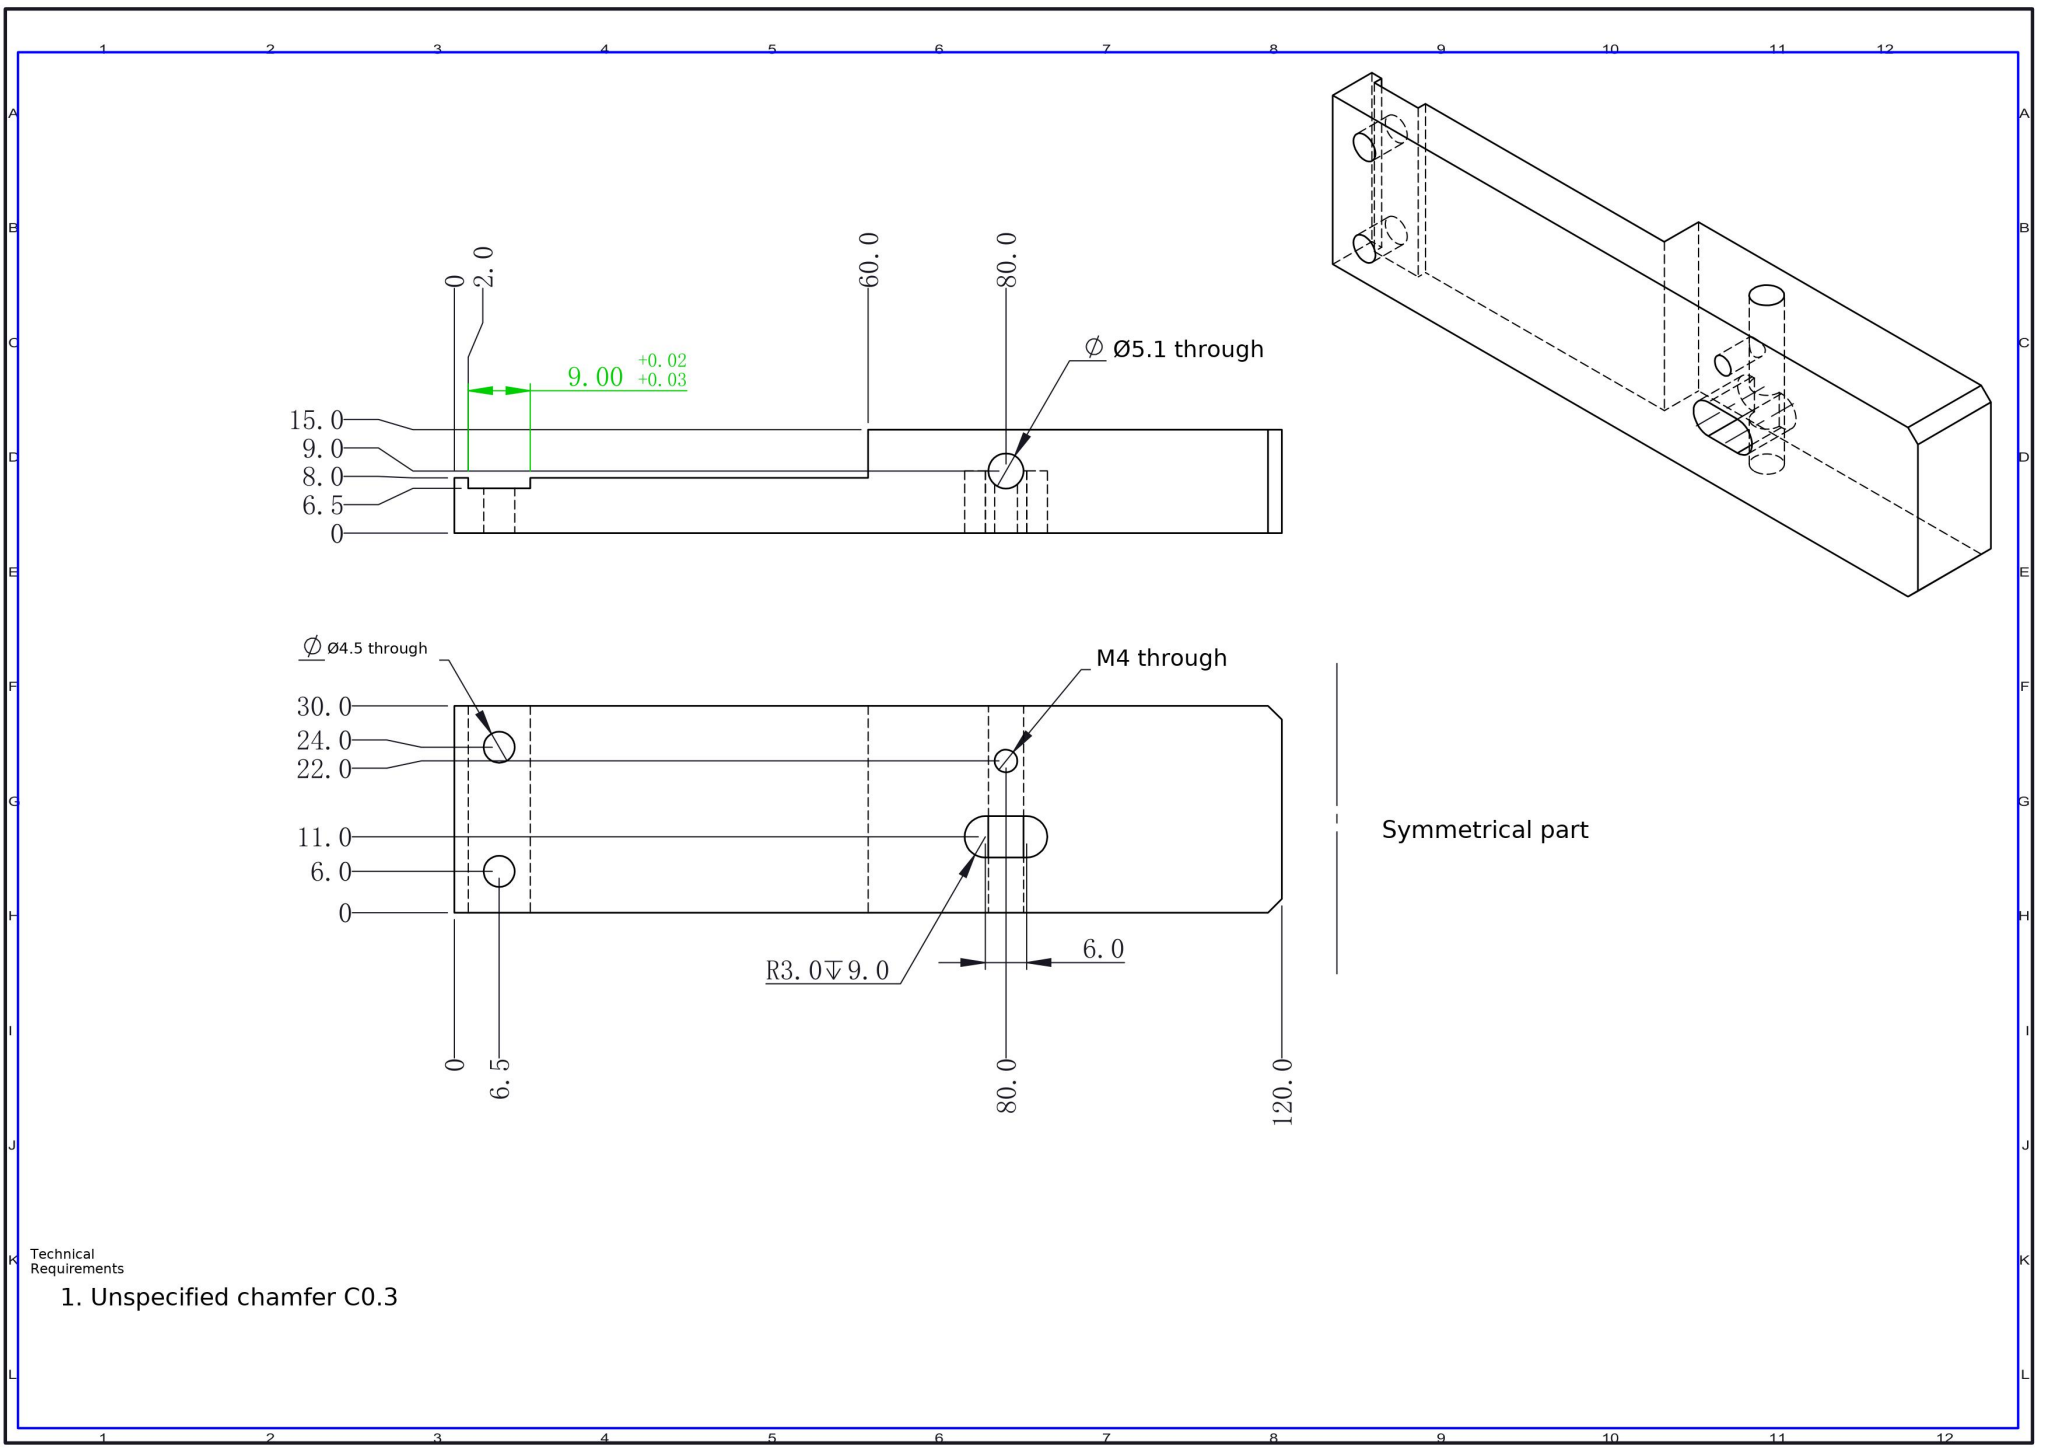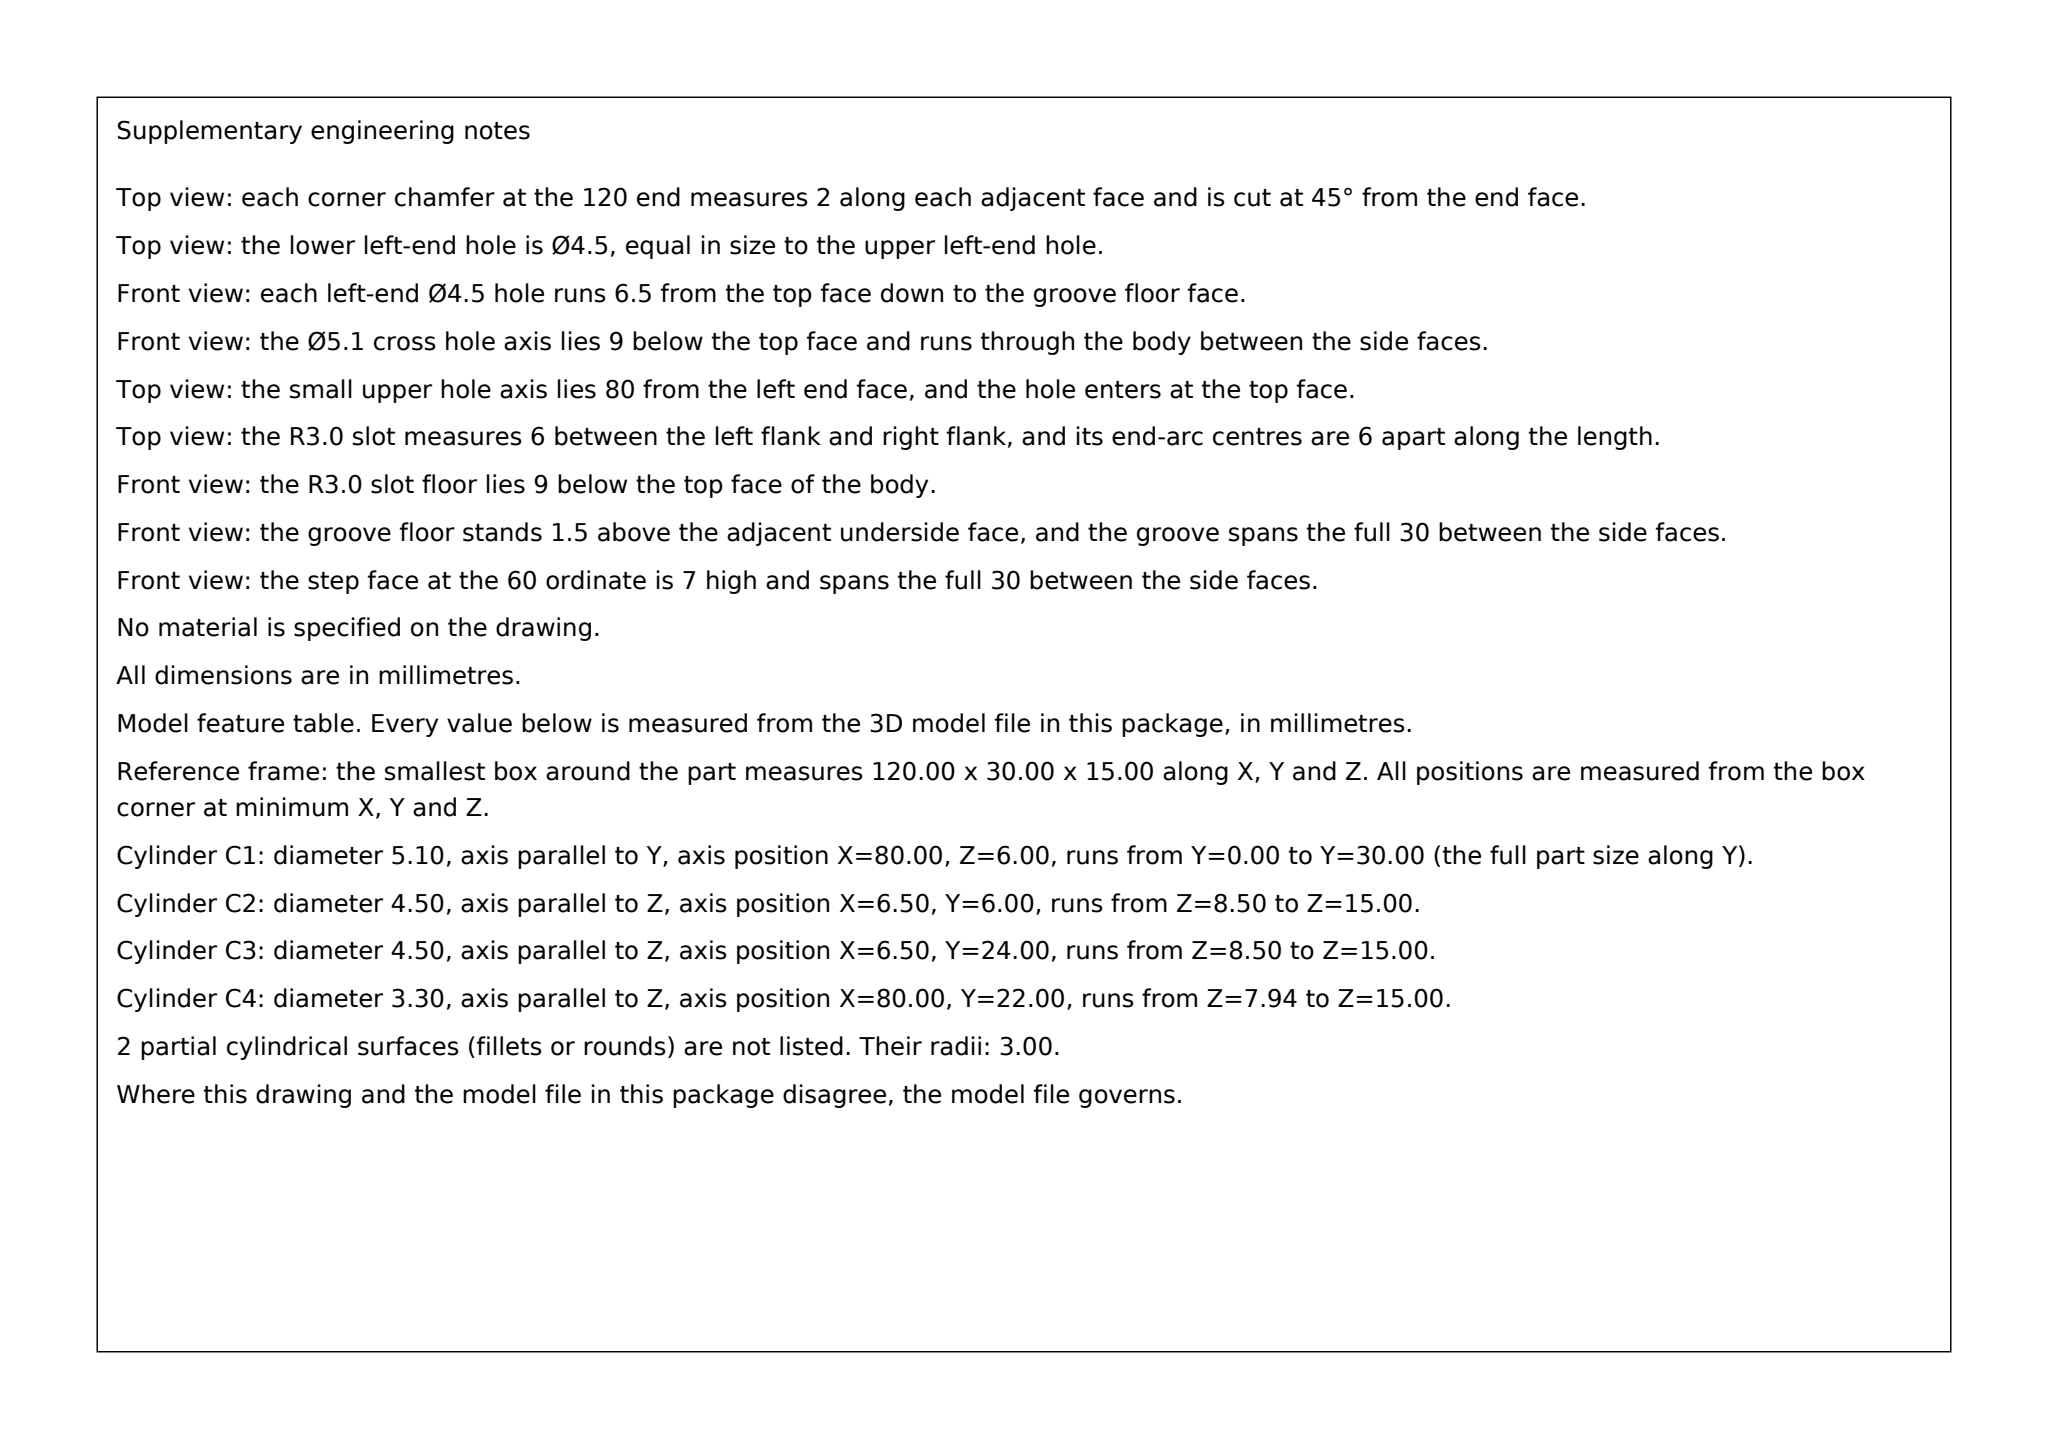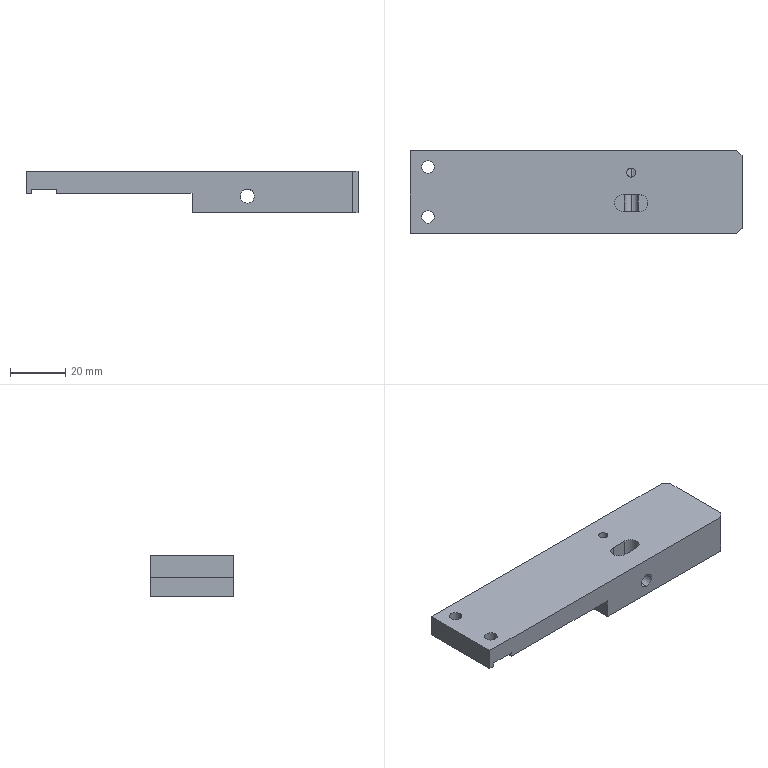Part | SolidWorks | mm | 1 solid | 29 faces | box 120 x 30 x 15 mm | volume 39542 mm3 | plane 18 | cylinder 11 | commonest cylinder face diameters 4.5 x4 6 x3 3.3 x2 5.1 x2
Drawing notes:
Ø5.1 THRU HOLE: AXIS 6.0 ABOVE BOTTOM FACE (Z0) | from the solid: cylinder dia 5.1, axis y, pos [x=80.0, z=6.0], length 30.0